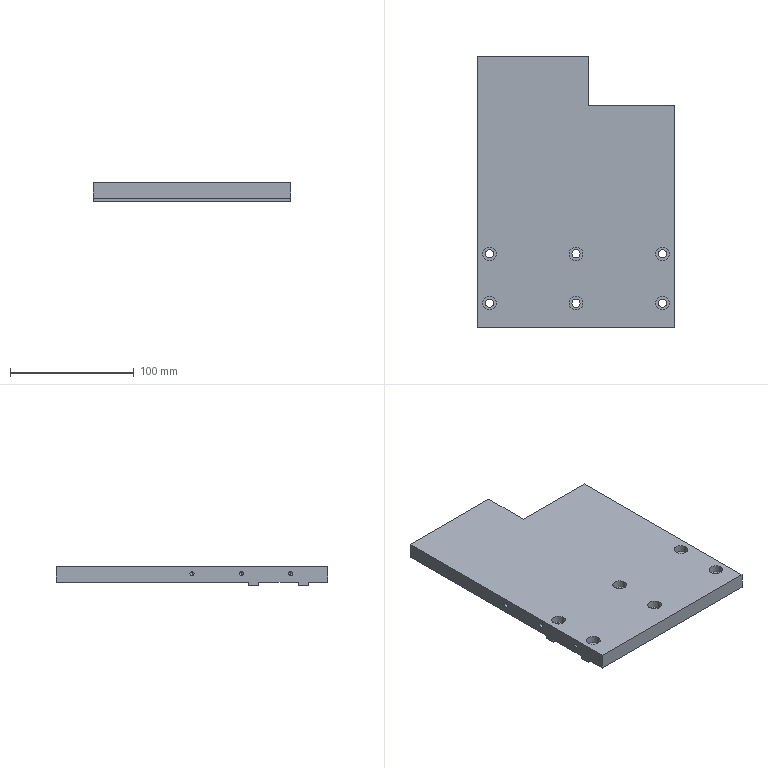Component | SolidWorks | Q1-A12-S21-Q4-10A-1 | 1 solid | 82 faces | box 160 x 220 x 15 mm | volume 405363 mm3 | cylinder 42 | plane 22 | cone 18 | commonest cylinder face diameters 3.3 x12 11 x12 6.6 x12 2.5 x6 | material White Plastic Steel POM
build123d program:
from build123d import *

# Parameters (mm, degrees)
SKETCH1_W                                            = 160
SKETCH1_H                                            = 220
BOSS_EXTRUDE1_DEPTH                                  = 15
CYLINDRICAL_COUNTERSUNK_HOLE_FOR_M6_SOCK_D           = 6.6
CYLINDRICAL_COUNTERSUNK_HOLE_FOR_M6_SOCK_CBORE_D     = 11
CYLINDRICAL_COUNTERSUNK_HOLE_FOR_M6_SOCK_CBORE_DEPTH = 6
SKETCH2_W                                            = 2.5
SKETCH2_H                                            = 15.9
SKETCH2_H_2                                          = 31.8
SKETCH2_H_3                                          = 155.9
CUT_EXTRUDE1_DEPTH                                   = 195.743
M4X0_7_TAPPED_HOLE1_D                                = 3.3
M4X0_7_TAPPED_HOLE1_DEPTH                            = 15
M4X0_7_TAPPED_HOLE1_TIP                              = 0.9914
M4X0_7_TAPPED_HOLE2_D                                = 3.3
M4X0_7_TAPPED_HOLE2_DEPTH                            = 15.5
M4X0_7_TAPPED_HOLE2_TIP                              = 0.9914
SKETCH10_W                                           = 70
SKETCH10_H                                           = 40
CUT_EXTRUDE2_DEPTH                                   = 137.839
M3X0_5_TAPPED_HOLE1_D                                = 2.5
M3X0_5_TAPPED_HOLE1_DEPTH                            = 8.5
M3X0_5_TAPPED_HOLE1_TIP                              = 0.7511


with BuildPart() as part:
    # Sketch1 → Boss-Extrude1 (new body)
    with BuildSketch(Plane.XY):
        Rectangle(SKETCH1_W, SKETCH1_H)
    extrude(amount=BOSS_EXTRUDE1_DEPTH)

    # Cylindrical Countersunk Hole for M6 Sock (through all)
    with Locations(Plane.XY.offset(15)):
        with Locations((70, -50), (70, -90), (-70, -50), (-70, -90), (0, -50), (0, -90)):
            CounterBoreHole(CYLINDRICAL_COUNTERSUNK_HOLE_FOR_M6_SOCK_D / 2, CYLINDRICAL_COUNTERSUNK_HOLE_FOR_M6_SOCK_CBORE_D / 2, CYLINDRICAL_COUNTERSUNK_HOLE_FOR_M6_SOCK_CBORE_DEPTH)

    # Sketch2 → Cut-Extrude1 (cut, through all)
    with BuildSketch(Plane(origin=(80, 0, 0), x_dir=(0, 0, -1), z_dir=(1, 0, 0))):
        with Locations((-1.25, -102.05)):
            Rectangle(SKETCH2_W, SKETCH2_H)
        with Locations((-1.25, -70)):
            Rectangle(SKETCH2_W, SKETCH2_H_2)
        with Locations((-1.25, 32.05)):
            Rectangle(SKETCH2_W, SKETCH2_H_3)
    extrude(amount=-CUT_EXTRUDE1_DEPTH, mode=Mode.SUBTRACT)

    # M4x0.7 Tapped Hole1
    with Locations(Plane(origin=(80, 0, 0), x_dir=(0, 0, -1), z_dir=(1, 0, 0))):
        with Locations((-9.5, 0), (-9.5, -40), (-9.5, -80)):
            Hole(M4X0_7_TAPPED_HOLE1_D / 2, depth=M4X0_7_TAPPED_HOLE1_DEPTH)
            with Locations((0, 0, -(M4X0_7_TAPPED_HOLE1_DEPTH + M4X0_7_TAPPED_HOLE1_TIP / 2))):  # 118° drill point
                Cone(0, M4X0_7_TAPPED_HOLE1_D / 2, M4X0_7_TAPPED_HOLE1_TIP, mode=Mode.SUBTRACT)

    # M4x0.7 Tapped Hole2
    with Locations(Plane.ZY.offset(80)):
        with Locations((9.5, 0), (9.5, -40), (9.5, -80)):
            Hole(M4X0_7_TAPPED_HOLE2_D / 2, depth=M4X0_7_TAPPED_HOLE2_DEPTH)
            with Locations((0, 0, -(M4X0_7_TAPPED_HOLE2_DEPTH + M4X0_7_TAPPED_HOLE2_TIP / 2))):  # 118° drill point
                Cone(0, M4X0_7_TAPPED_HOLE2_D / 2, M4X0_7_TAPPED_HOLE2_TIP, mode=Mode.SUBTRACT)

    # Sketch10 → Cut-Extrude2 (cut, through all)
    with BuildSketch(Plane.XY.offset(15)):
        with Locations((45, 90)):
            Rectangle(SKETCH10_W, SKETCH10_H)
    extrude(amount=-CUT_EXTRUDE2_DEPTH, mode=Mode.SUBTRACT)

    # M3x0.5 Tapped Hole1
    with Locations(Plane(origin=(0, 110, 0), x_dir=(1, 0, 0), z_dir=(0, 1, 0))):
        with Locations((0, -10), (-30, -10), (-70, -10)):
            Hole(M3X0_5_TAPPED_HOLE1_D / 2, depth=M3X0_5_TAPPED_HOLE1_DEPTH)
            with Locations((0, 0, -(M3X0_5_TAPPED_HOLE1_DEPTH + M3X0_5_TAPPED_HOLE1_TIP / 2))):  # 118° drill point
                Cone(0, M3X0_5_TAPPED_HOLE1_D / 2, M3X0_5_TAPPED_HOLE1_TIP, mode=Mode.SUBTRACT)


solid = part.part

# Placed as in the assembly
solid = solid.moved(Location((298.5, 70, 147.5), (0, 0, 0)))